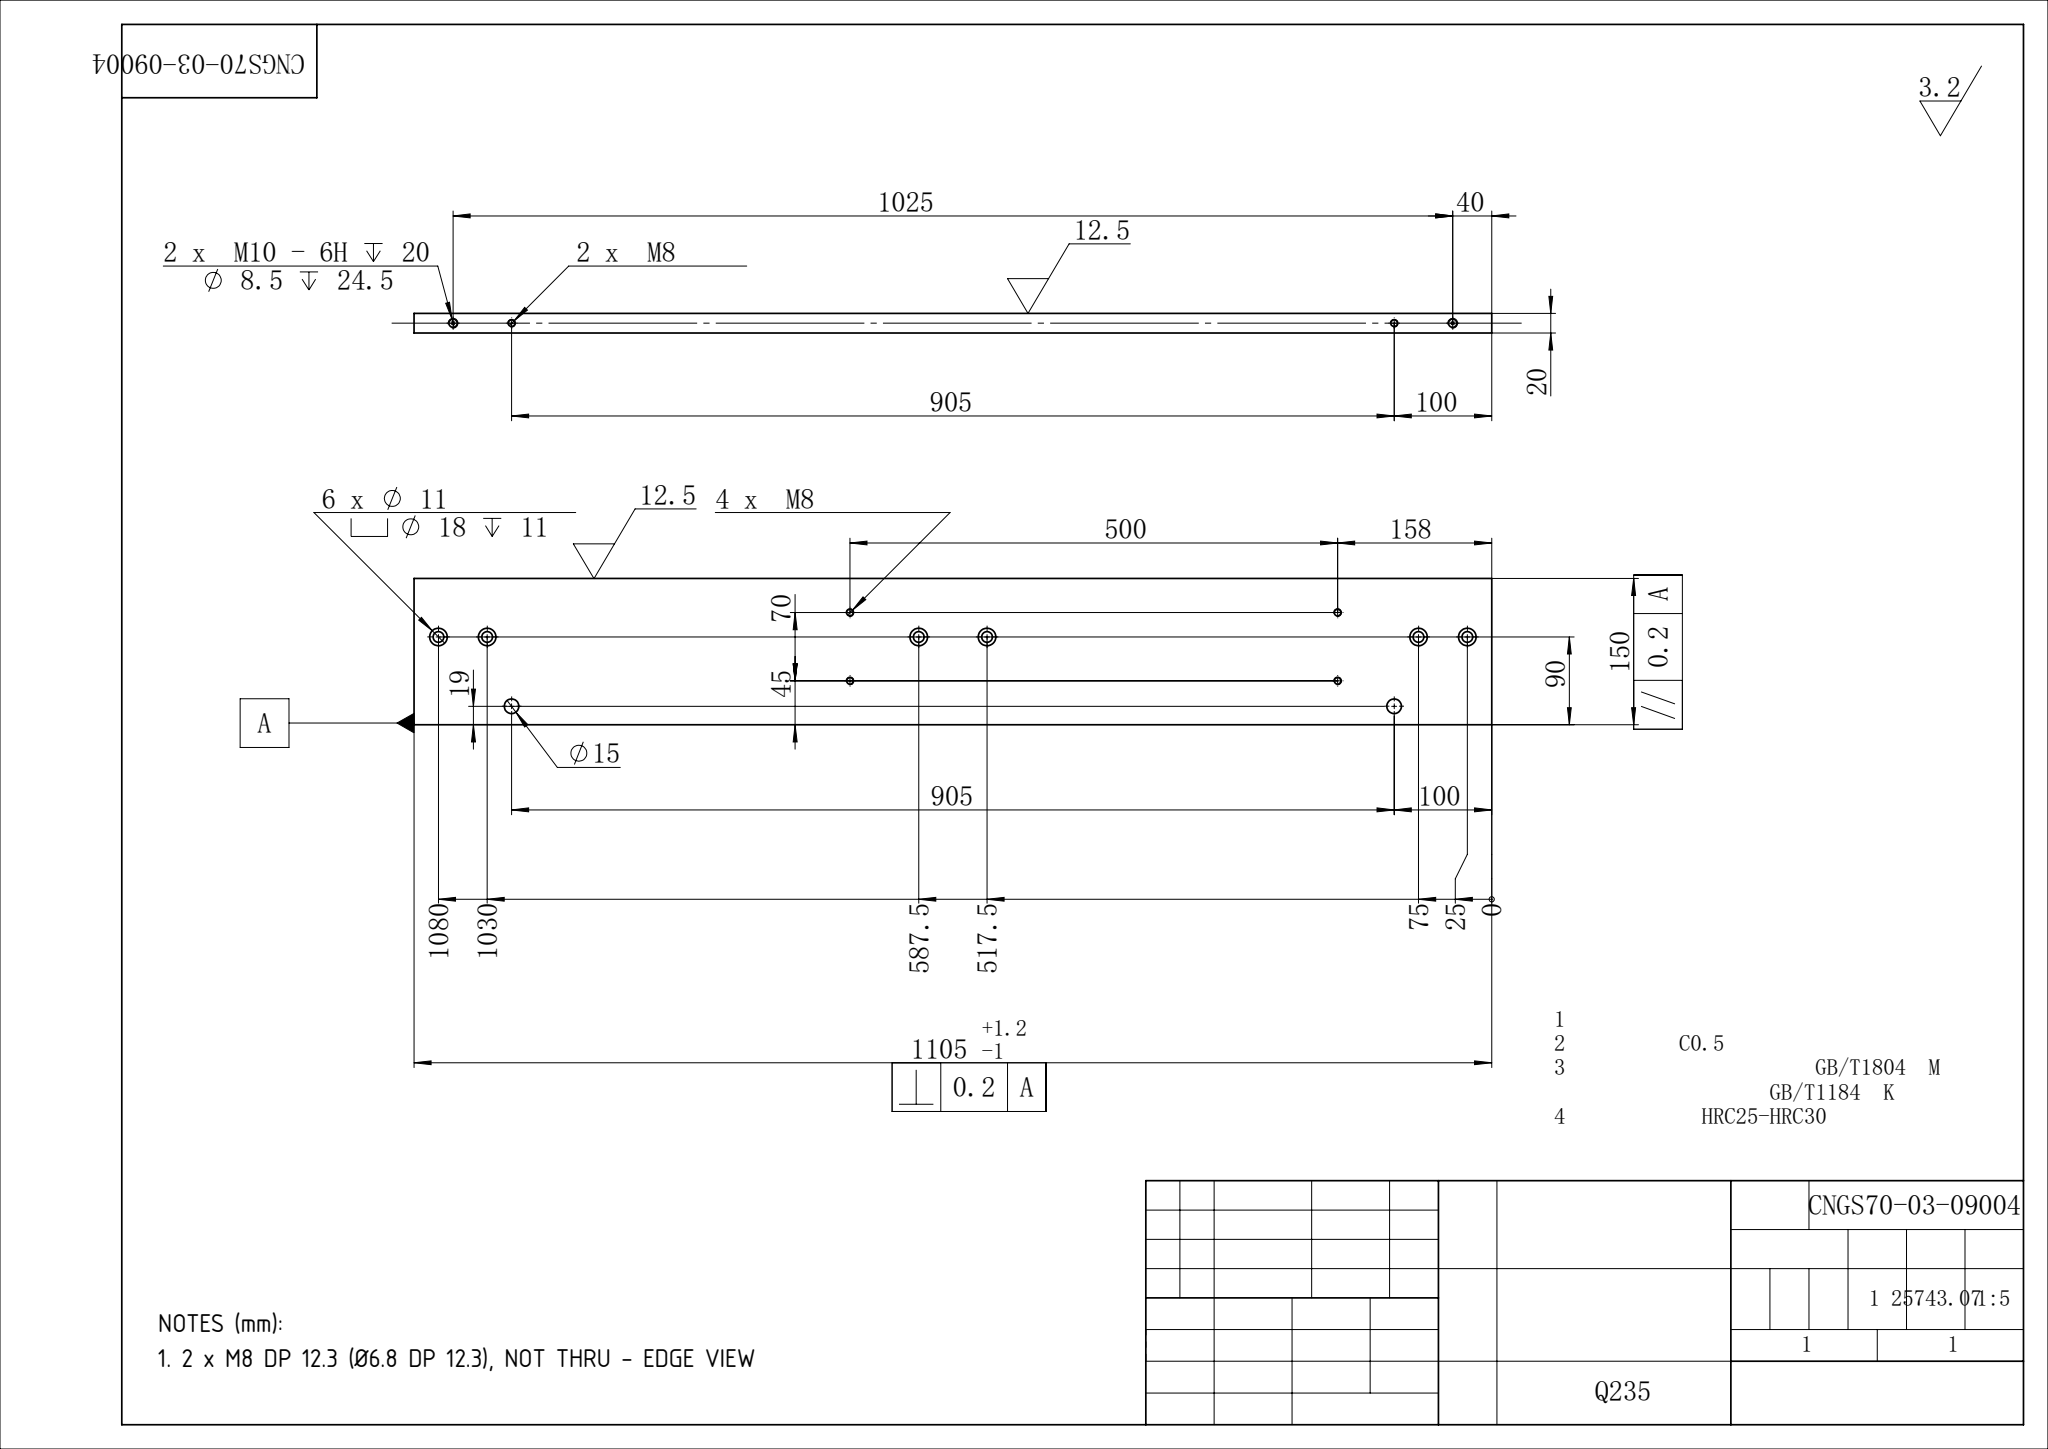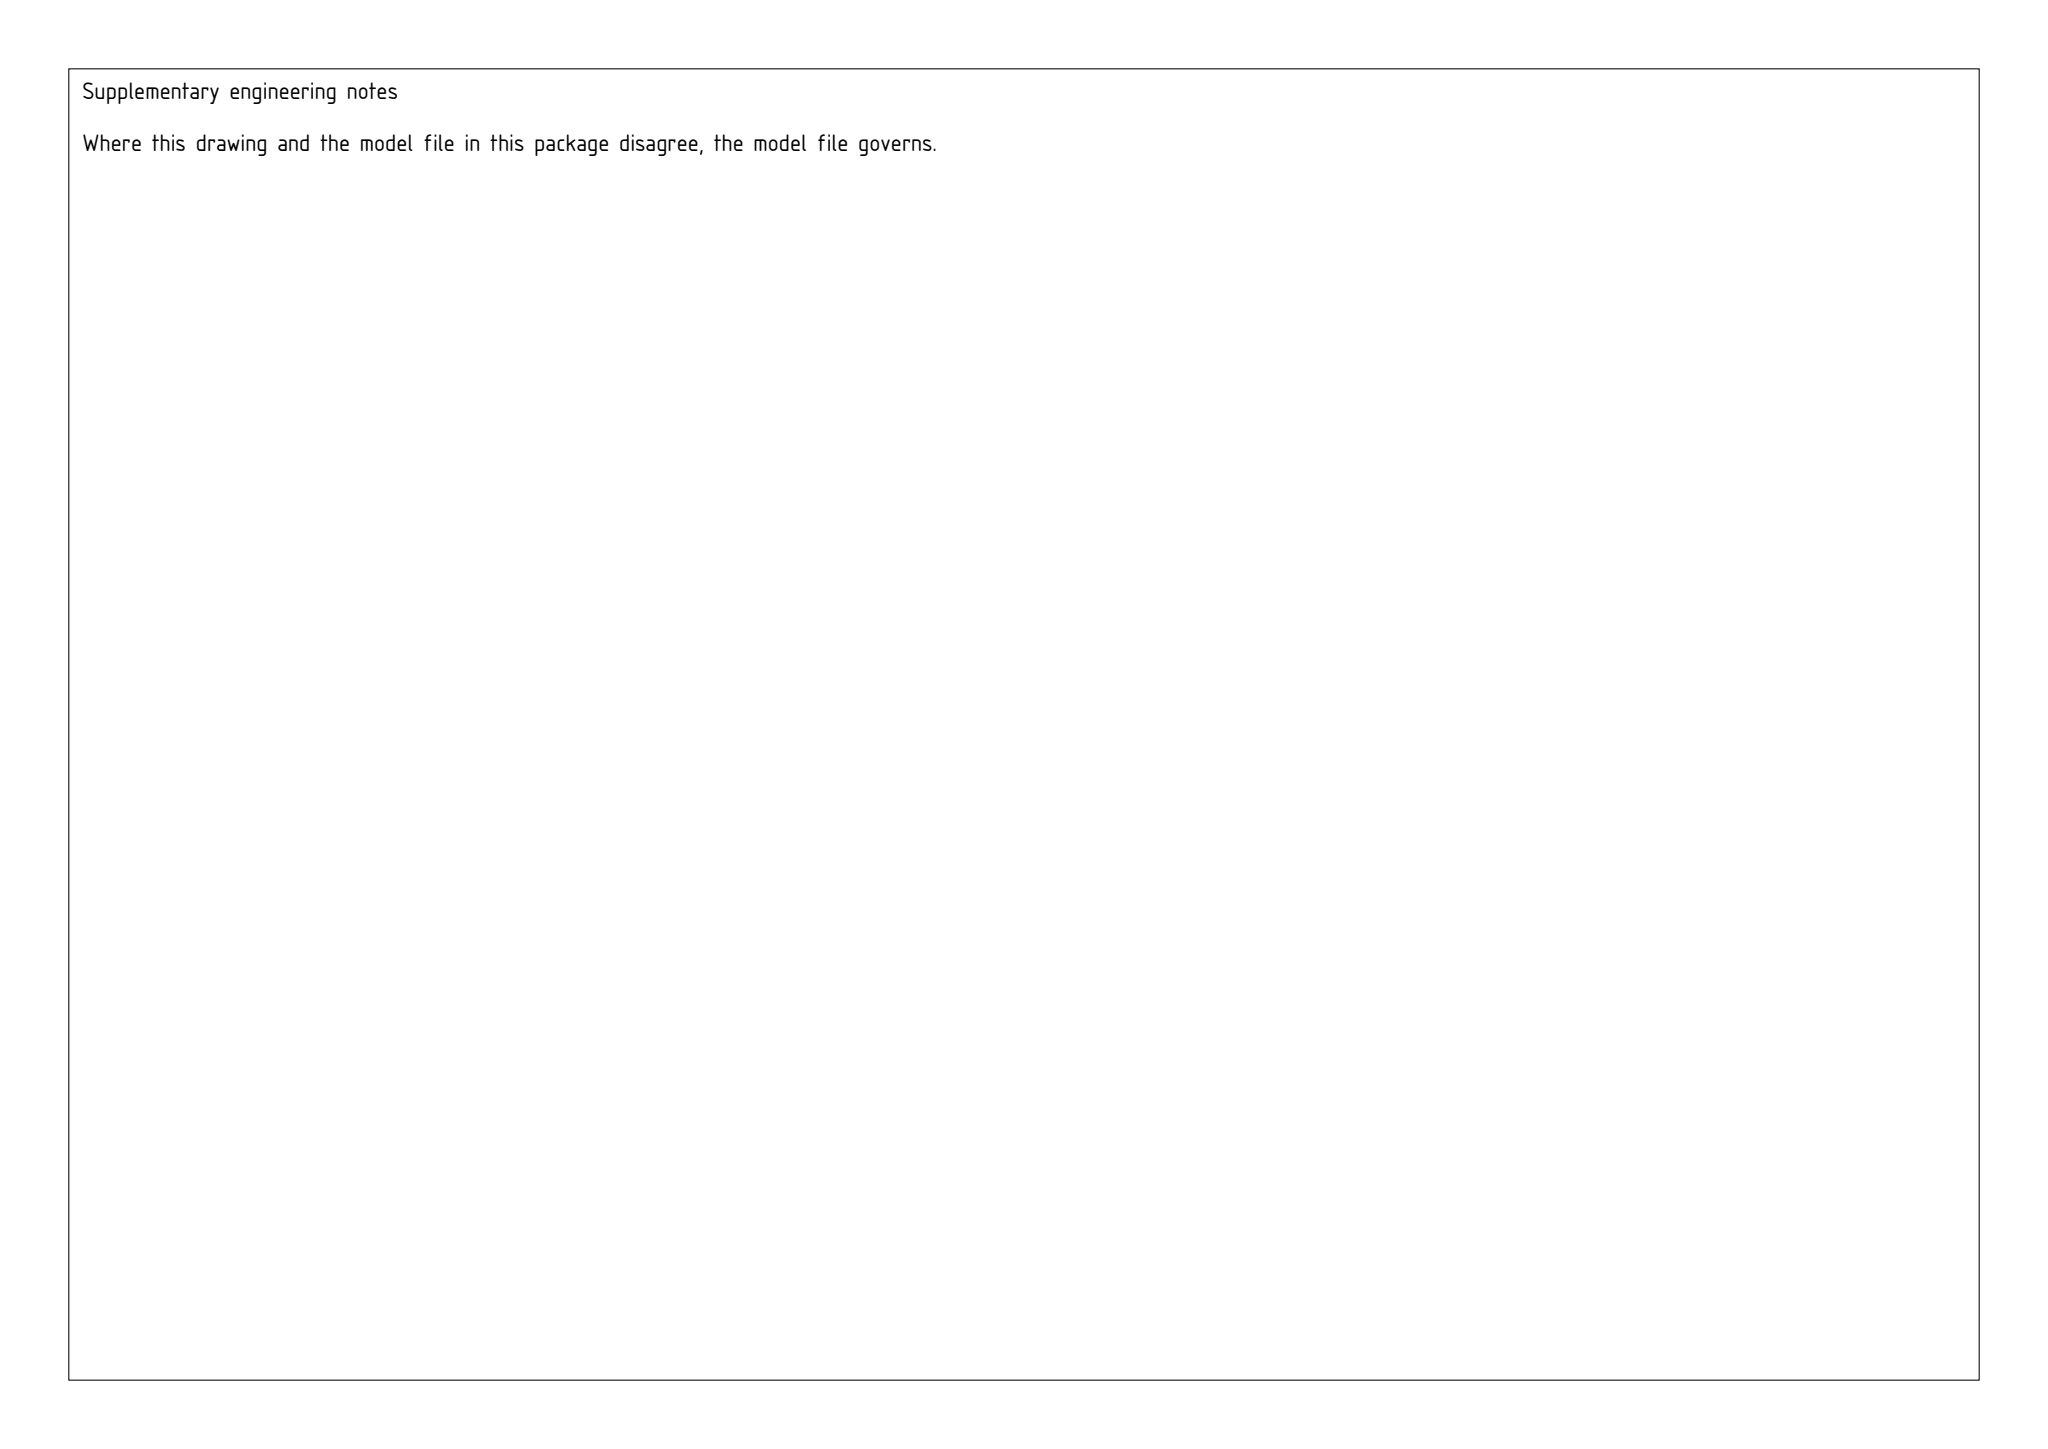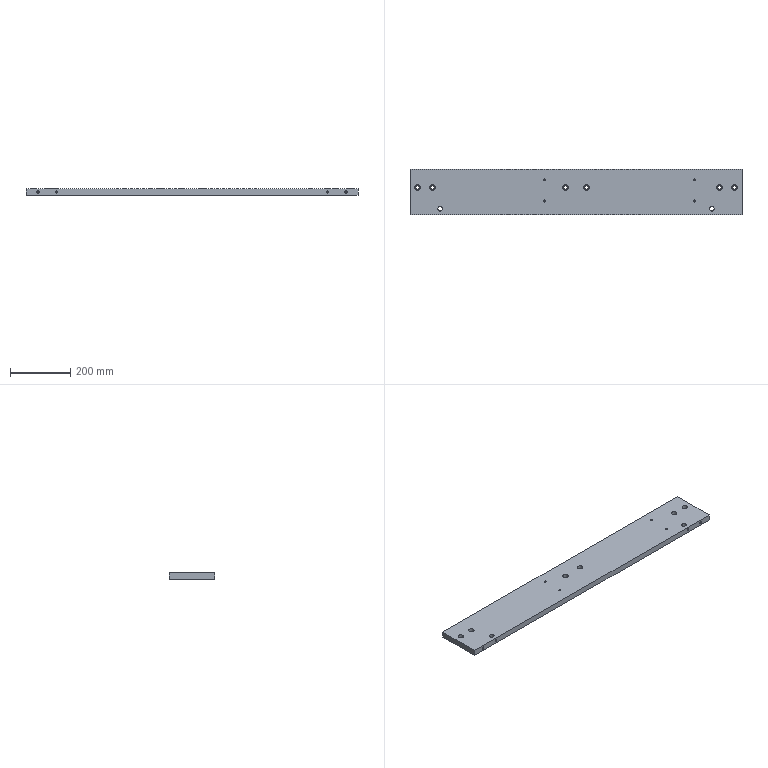Part | SolidWorks | mm | 1 solid | 60 faces | box 1105 x 150 x 20 mm | volume 3279372 mm3 | cylinder 44 | plane 12 | cone 4 | commonest cylinder face diameters 6.8 x12 18 x12 11 x12 8.5 x4 15 x4
Drawing notes:
2 x M8 DP 12.3 (Ø6.8 DP 12.3), NOT THRU - EDGE VIEW | from the solid: cylinders dia 6.8 axis y at x=100 & x=1005, z=10, length 12.32 (blind, bbox y=150)